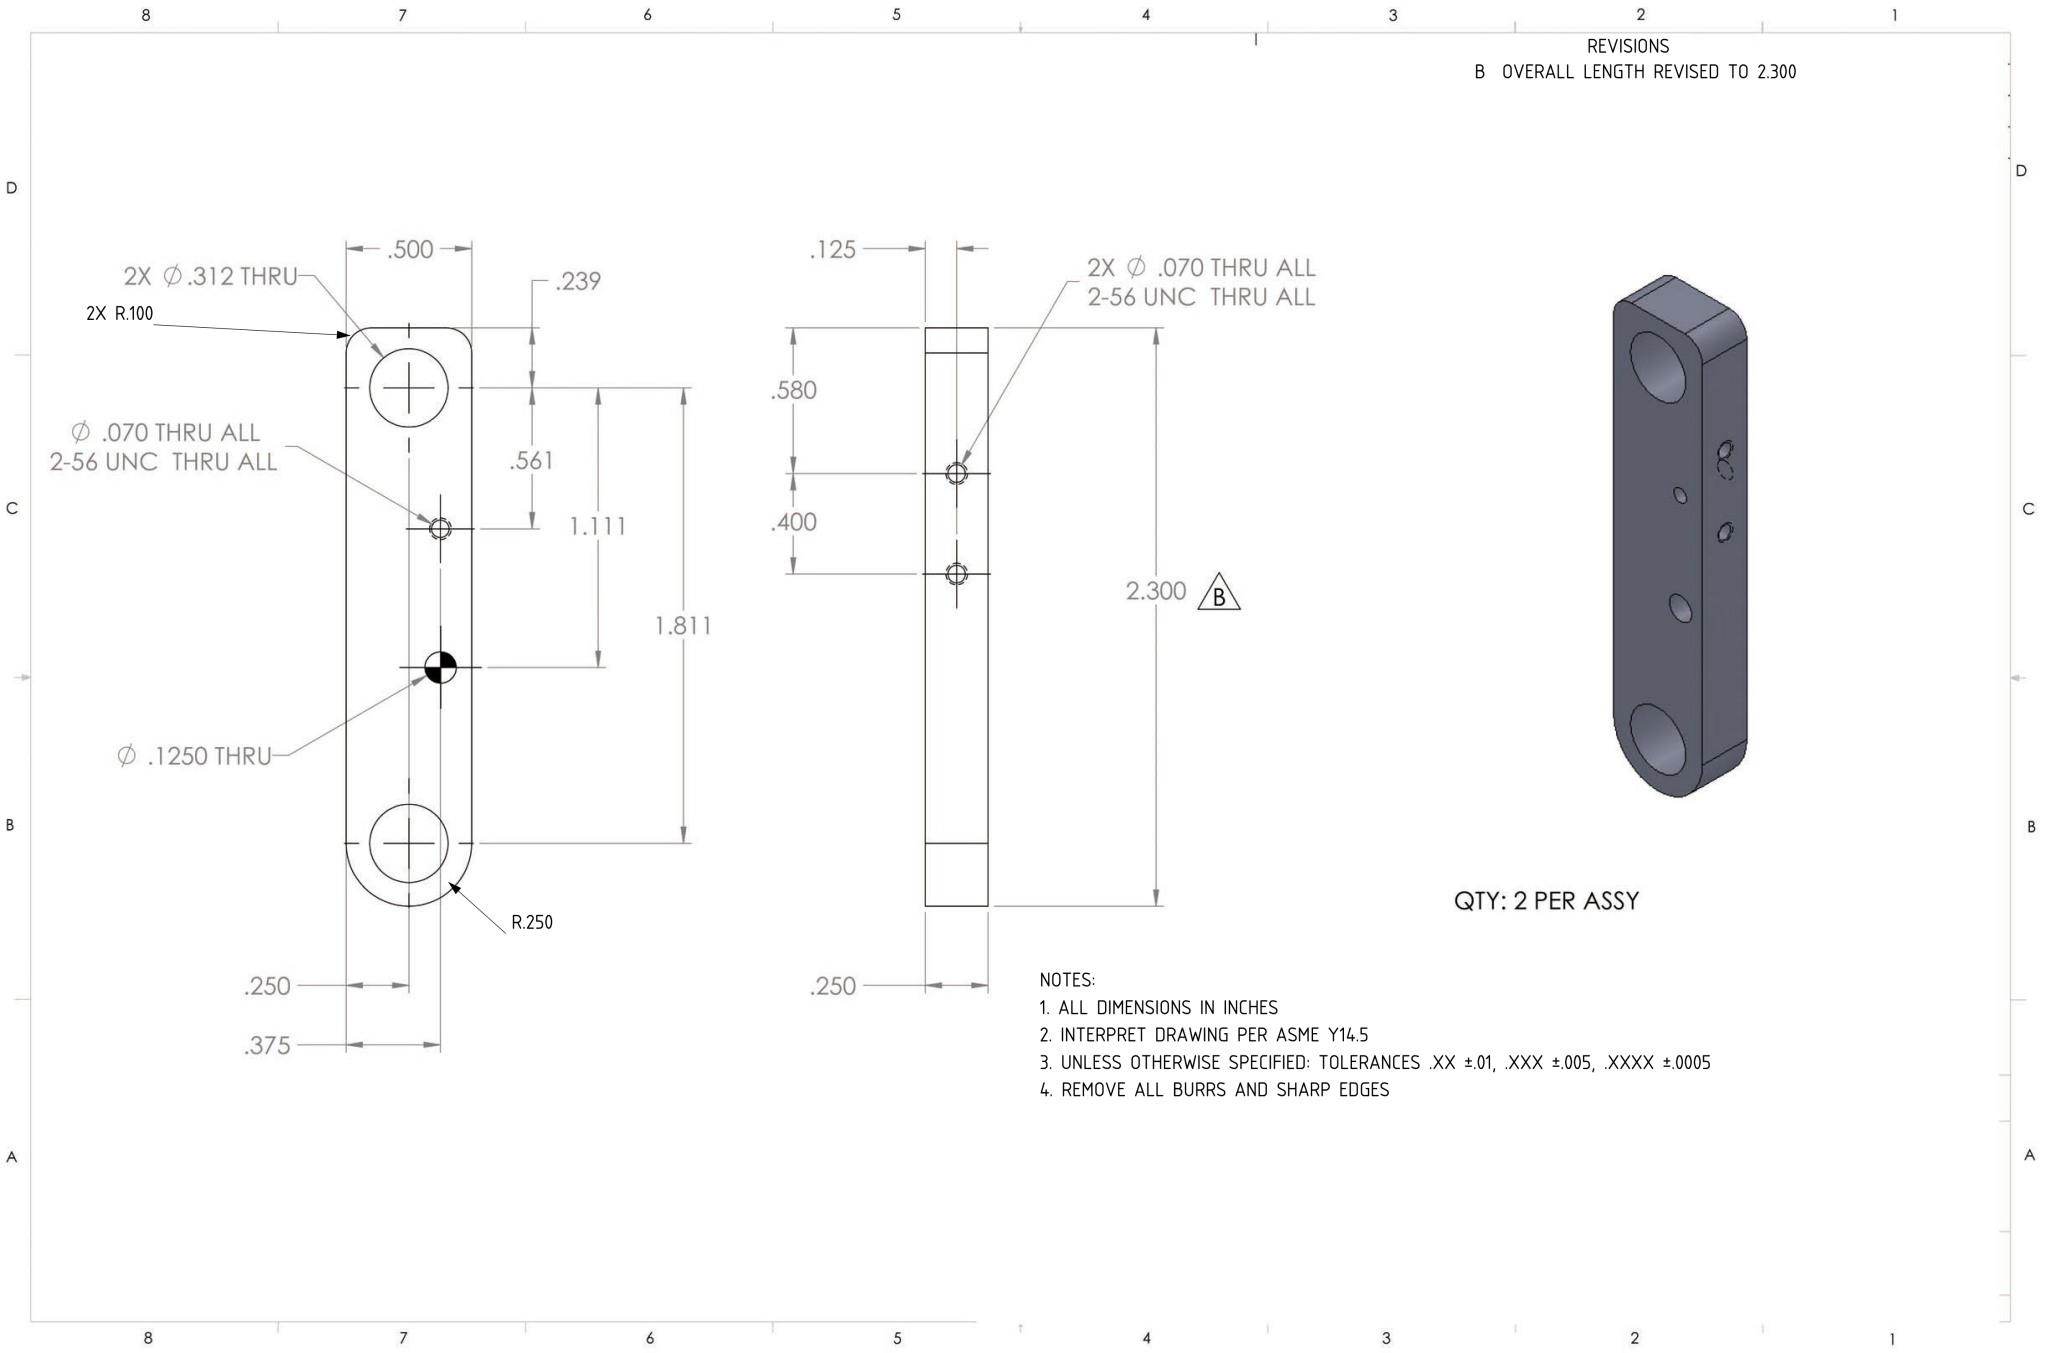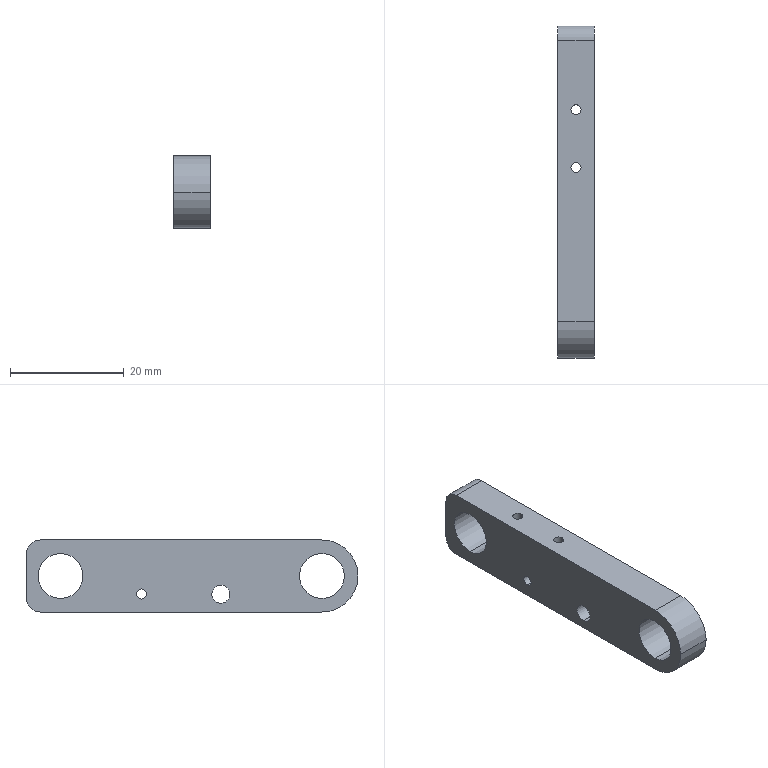Part | NX | drawing in inches | 1 solid | 21 faces | box 6.35 x 58.42 x 12.7 mm | volume 3828 mm3 | cylinder 16 | plane 5 | commonest cylinder face diameters 1.778 x6 7.925 x4 3.175 x2 5.08 x2 12.7 x2
STEP:
#1=COLOUR_RGB('',0.7922,0.8196,0.9333);
#2=FILL_AREA_STYLE_COLOUR('',#1);
#3=FILL_AREA_STYLE('',(#2));
#4=SURFACE_STYLE_FILL_AREA(#3);
#5=SURFACE_SIDE_STYLE('',(#4));
#6=SURFACE_STYLE_USAGE(.BOTH.,#5);
#7=PRESENTATION_STYLE_ASSIGNMENT((#6));
#8=CARTESIAN_POINT('',(-0.09,1.47,0.25));
#9=VERTEX_POINT('',#8);
#10=CARTESIAN_POINT('',(-0.09,1.47,-0.25));
#11=VERTEX_POINT('',#10);
#12=CARTESIAN_POINT('',(-0.09,1.47,-0.25));
#13=DIRECTION('',(0.,0.,-1.));
#14=VECTOR('',#13,39.37);
#15=LINE('',#12,#14);
#16=EDGE_CURVE('',#9,#11,#15,.T.);
#17=ORIENTED_EDGE('',*,*,#16,.F.);
#18=CARTESIAN_POINT('',(-0.16,1.47,0.25));
#19=VERTEX_POINT('',#18);
#20=CARTESIAN_POINT('',(-0.125,1.47,0.25));
#21=DIRECTION('',(0.,0.,-1.));
#22=DIRECTION('',(-1.,0.,0.));
#23=AXIS2_PLACEMENT_3D('',#20,#21,#22);
#24=CIRCLE('',#23,0.035);
#25=EDGE_CURVE('',#19,#9,#24,.T.);
#26=ORIENTED_EDGE('',*,*,#25,.F.);
#27=CARTESIAN_POINT('',(-0.16,1.47,-0.25));
#28=VERTEX_POINT('',#27);
#29=CARTESIAN_POINT('',(-0.16,1.47,-0.25));
#30=DIRECTION('',(0.,0.,-1.));
#31=VECTOR('',#30,39.37);
#32=LINE('',#29,#31);
#33=EDGE_CURVE('',#19,#28,#32,.T.);
#34=ORIENTED_EDGE('',*,*,#33,.T.);
#35=CARTESIAN_POINT('',(-0.125,1.47,-0.25));
#36=DIRECTION('',(0.,0.,-1.));
#37=DIRECTION('',(-1.,0.,0.));
#38=AXIS2_PLACEMENT_3D('',#35,#36,#37);
#39=CIRCLE('',#38,0.035);
#40=EDGE_CURVE('',#28,#11,#39,.T.);
#41=ORIENTED_EDGE('',*,*,#40,.T.);
#42=EDGE_LOOP('',(#17,#26,#34,#41));
#43=FACE_OUTER_BOUND('',#42,.T.);
#44=CARTESIAN_POINT('',(-0.125,1.47,-0.25));
#45=DIRECTION('',(0.,0.,-1.));
#46=DIRECTION('',(-1.,0.,0.));
#47=AXIS2_PLACEMENT_3D('',#44,#45,#46);
#48=CYLINDRICAL_SURFACE('',#47,0.035);
#49=ADVANCED_FACE('',(#43),#48,.F.);
#50=STYLED_ITEM('',(#7),#49);
#51=PRESENTATION_LAYER_ASSIGNMENT('','',(#50));
#52=COLOUR_RGB('',0.7922,0.8196,0.9333);
#53=FILL_AREA_STYLE_COLOUR('',#52);
#54=FILL_AREA_STYLE('',(#53));
#55=SURFACE_STYLE_FILL_AREA(#54);
#56=SURFACE_SIDE_STYLE('',(#55));
#57=SURFACE_STYLE_USAGE(.BOTH.,#56);
#58=PRESENTATION_STYLE_ASSIGNMENT((#57));
#59=CARTESIAN_POINT('',(0.,1.25,-0.16));
#60=VERTEX_POINT('',#59);
#61=CARTESIAN_POINT('',(0.,1.25,-0.09));
#62=VERTEX_POINT('',#61);
#63=CARTESIAN_POINT('',(0.,1.25,-0.125));
#64=DIRECTION('',(-1.,0.,0.));
#65=DIRECTION('',(0.,0.,1.));
#66=AXIS2_PLACEMENT_3D('',#63,#64,#65);
#67=CIRCLE('',#66,0.035);
#68=EDGE_CURVE('',#60,#62,#67,.T.);
#69=ORIENTED_EDGE('',*,*,#68,.F.);
#70=CARTESIAN_POINT('',(-0.25,1.25,-0.16));
#71=VERTEX_POINT('',#70);
#72=CARTESIAN_POINT('',(-0.25,1.25,-0.16));
#73=DIRECTION('',(-1.,0.,0.));
#74=VECTOR('',#73,39.37);
#75=LINE('',#72,#74);
#76=EDGE_CURVE('',#60,#71,#75,.T.);
#77=ORIENTED_EDGE('',*,*,#76,.T.);
#78=CARTESIAN_POINT('',(-0.25,1.25,-0.09));
#79=VERTEX_POINT('',#78);
#80=CARTESIAN_POINT('',(-0.25,1.25,-0.125));
#81=DIRECTION('',(-1.,0.,0.));
#82=DIRECTION('',(0.,0.,1.));
#83=AXIS2_PLACEMENT_3D('',#80,#81,#82);
#84=CIRCLE('',#83,0.035);
#85=EDGE_CURVE('',#71,#79,#84,.T.);
#86=ORIENTED_EDGE('',*,*,#85,.T.);
#87=CARTESIAN_POINT('',(-0.25,1.25,-0.09));
#88=DIRECTION('',(-1.,0.,0.));
#89=VECTOR('',#88,39.37);
#90=LINE('',#87,#89);
#91=EDGE_CURVE('',#62,#79,#90,.T.);
#92=ORIENTED_EDGE('',*,*,#91,.F.);
#93=EDGE_LOOP('',(#69,#77,#86,#92));
#94=FACE_OUTER_BOUND('',#93,.T.);
#95=CARTESIAN_POINT('',(-0.25,1.25,-0.125));
#96=DIRECTION('',(-1.,0.,0.));
#97=DIRECTION('',(0.,0.,1.));
#98=AXIS2_PLACEMENT_3D('',#95,#96,#97);
#99=CYLINDRICAL_SURFACE('',#98,0.035);
#100=ADVANCED_FACE('',(#94),#99,.F.);
#101=CARTESIAN_POINT('',(-0.25,0.7,-0.1886));
#102=VERTEX_POINT('',#101);
#103=CARTESIAN_POINT('',(-0.25,0.7,-0.06365));
#104=VERTEX_POINT('',#103);
#105=CARTESIAN_POINT('',(-0.25,0.7,-0.1261));
#106=DIRECTION('',(-1.,0.,0.));
#107=DIRECTION('',(0.,0.,1.));
#108=AXIS2_PLACEMENT_3D('',#105,#106,#107);
#109=CIRCLE('',#108,0.0625);
#110=EDGE_CURVE('',#102,#104,#109,.T.);
#111=ORIENTED_EDGE('',*,*,#110,.T.);
#112=CARTESIAN_POINT('',(0.,0.7,-0.06365));
#113=VERTEX_POINT('',#112);
#114=CARTESIAN_POINT('',(0.,0.7,-0.06365));
#115=DIRECTION('',(1.,0.,0.));
#116=VECTOR('',#115,39.37);
#117=LINE('',#114,#116);
#118=EDGE_CURVE('',#104,#113,#117,.T.);
#119=ORIENTED_EDGE('',*,*,#118,.T.);
#120=CARTESIAN_POINT('',(0.,0.7,-0.1886));
#121=VERTEX_POINT('',#120);
#122=CARTESIAN_POINT('',(0.,0.7,-0.1261));
#123=DIRECTION('',(1.,0.,0.));
#124=DIRECTION('',(0.,0.,-1.));
#125=AXIS2_PLACEMENT_3D('',#122,#123,#124);
#126=CIRCLE('',#125,0.0625);
#127=EDGE_CURVE('',#113,#121,#126,.T.);
#128=ORIENTED_EDGE('',*,*,#127,.T.);
#129=CARTESIAN_POINT('',(0.,0.7,-0.1886));
#130=DIRECTION('',(1.,0.,0.));
#131=VECTOR('',#130,39.37);
#132=LINE('',#129,#131);
#133=EDGE_CURVE('',#102,#121,#132,.T.);
#134=ORIENTED_EDGE('',*,*,#133,.F.);
#135=EDGE_LOOP('',(#111,#119,#128,#134));
#136=FACE_OUTER_BOUND('',#135,.T.);
#137=CARTESIAN_POINT('',(0.,0.7,-0.1261));
#138=DIRECTION('',(1.,0.,0.));
#139=DIRECTION('',(0.,0.,-1.));
#140=AXIS2_PLACEMENT_3D('',#137,#138,#139);
#141=CYLINDRICAL_SURFACE('',#140,0.0625);
#142=ADVANCED_FACE('',(#136),#141,.F.);
#143=CARTESIAN_POINT('',(-0.125,1.47,0.25));
#144=DIRECTION('',(0.,0.,-1.));
#145=DIRECTION('',(-1.,0.,0.));
#146=AXIS2_PLACEMENT_3D('',#143,#144,#145);
#147=CIRCLE('',#146,0.035);
#148=EDGE_CURVE('',#9,#19,#147,.T.);
#149=ORIENTED_EDGE('',*,*,#148,.F.);
#150=ORIENTED_EDGE('',*,*,#16,.T.);
#151=CARTESIAN_POINT('',(-0.125,1.47,-0.25));
#152=DIRECTION('',(0.,0.,-1.));
#153=DIRECTION('',(-1.,0.,0.));
#154=AXIS2_PLACEMENT_3D('',#151,#152,#153);
#155=CIRCLE('',#154,0.035);
#156=EDGE_CURVE('',#11,#28,#155,.T.);
#157=ORIENTED_EDGE('',*,*,#156,.T.);
#158=ORIENTED_EDGE('',*,*,#33,.F.);
#159=EDGE_LOOP('',(#149,#150,#157,#158));
#160=FACE_OUTER_BOUND('',#159,.T.);
#161=CARTESIAN_POINT('',(-0.125,1.47,-0.25));
#162=DIRECTION('',(0.,0.,-1.));
#163=DIRECTION('',(-1.,0.,0.));
#164=AXIS2_PLACEMENT_3D('',#161,#162,#163);
#165=CYLINDRICAL_SURFACE('',#164,0.035);
#166=ADVANCED_FACE('',(#160),#165,.F.);
#167=CARTESIAN_POINT('',(-0.09,1.07,0.25));
#168=VERTEX_POINT('',#167);
#169=CARTESIAN_POINT('',(-0.16,1.07,0.25));
#170=VERTEX_POINT('',#169);
#171=CARTESIAN_POINT('',(-0.125,1.07,0.25));
#172=DIRECTION('',(0.,0.,-1.));
#173=DIRECTION('',(-1.,0.,0.));
#174=AXIS2_PLACEMENT_3D('',#171,#172,#173);
#175=CIRCLE('',#174,0.035);
#176=EDGE_CURVE('',#168,#170,#175,.T.);
#177=ORIENTED_EDGE('',*,*,#176,.F.);
#178=CARTESIAN_POINT('',(-0.09,1.07,-0.25));
#179=VERTEX_POINT('',#178);
#180=CARTESIAN_POINT('',(-0.09,1.07,-0.25));
#181=DIRECTION('',(0.,0.,-1.));
#182=VECTOR('',#181,39.37);
#183=LINE('',#180,#182);
#184=EDGE_CURVE('',#168,#179,#183,.T.);
#185=ORIENTED_EDGE('',*,*,#184,.T.);
#186=CARTESIAN_POINT('',(-0.16,1.07,-0.25));
#187=VERTEX_POINT('',#186);
#188=CARTESIAN_POINT('',(-0.125,1.07,-0.25));
#189=DIRECTION('',(0.,0.,-1.));
#190=DIRECTION('',(-1.,0.,0.));
#191=AXIS2_PLACEMENT_3D('',#188,#189,#190);
#192=CIRCLE('',#191,0.035);
#193=EDGE_CURVE('',#179,#187,#192,.T.);
#194=ORIENTED_EDGE('',*,*,#193,.T.);
#195=CARTESIAN_POINT('',(-0.16,1.07,-0.25));
#196=DIRECTION('',(0.,0.,-1.));
#197=VECTOR('',#196,39.37);
#198=LINE('',#195,#197);
#199=EDGE_CURVE('',#170,#187,#198,.T.);
#200=ORIENTED_EDGE('',*,*,#199,.F.);
#201=EDGE_LOOP('',(#177,#185,#194,#200));
#202=FACE_OUTER_BOUND('',#201,.T.);
#203=CARTESIAN_POINT('',(-0.125,1.07,-0.25));
#204=DIRECTION('',(0.,0.,-1.));
#205=DIRECTION('',(-1.,0.,0.));
#206=AXIS2_PLACEMENT_3D('',#203,#204,#205);
#207=CYLINDRICAL_SURFACE('',#206,0.035);
#208=ADVANCED_FACE('',(#202),#207,.F.);
#209=CARTESIAN_POINT('',(-0.25,1.811,0.156));
#210=VERTEX_POINT('',#209);
#211=CARTESIAN_POINT('',(-0.25,1.811,-0.156));
#212=VERTEX_POINT('',#211);
#213=CARTESIAN_POINT('',(-0.25,1.811,0.));
#214=DIRECTION('',(1.,0.,0.));
#215=DIRECTION('',(0.,0.,1.));
#216=AXIS2_PLACEMENT_3D('',#213,#214,#215);
#217=CIRCLE('',#216,0.156);
#218=EDGE_CURVE('',#210,#212,#217,.T.);
#219=ORIENTED_EDGE('',*,*,#218,.F.);
#220=CARTESIAN_POINT('',(0.,1.811,0.156));
#221=VERTEX_POINT('',#220);
#222=CARTESIAN_POINT('',(-0.25,1.811,0.156));
#223=DIRECTION('',(1.,0.,0.));
#224=VECTOR('',#223,39.37);
#225=LINE('',#222,#224);
#226=EDGE_CURVE('',#210,#221,#225,.T.);
#227=ORIENTED_EDGE('',*,*,#226,.T.);
#228=CARTESIAN_POINT('',(0.,1.811,-0.156));
#229=VERTEX_POINT('',#228);
#230=CARTESIAN_POINT('',(0.,1.811,0.));
#231=DIRECTION('',(1.,0.,0.));
#232=DIRECTION('',(0.,0.,-1.));
#233=AXIS2_PLACEMENT_3D('',#230,#231,#232);
#234=CIRCLE('',#233,0.156);
#235=EDGE_CURVE('',#221,#229,#234,.T.);
#236=ORIENTED_EDGE('',*,*,#235,.T.);
#237=CARTESIAN_POINT('',(-0.25,1.811,-0.156));
#238=DIRECTION('',(1.,0.,0.));
#239=VECTOR('',#238,39.37);
#240=LINE('',#237,#239);
#241=EDGE_CURVE('',#212,#229,#240,.T.);
#242=ORIENTED_EDGE('',*,*,#241,.F.);
#243=EDGE_LOOP('',(#219,#227,#236,#242));
#244=FACE_OUTER_BOUND('',#243,.T.);
#245=CARTESIAN_POINT('',(-0.25,1.811,0.));
#246=DIRECTION('',(1.,0.,0.));
#247=DIRECTION('',(0.,0.,-1.));
#248=AXIS2_PLACEMENT_3D('',#245,#246,#247);
#249=CYLINDRICAL_SURFACE('',#248,0.156);
#250=ADVANCED_FACE('',(#244),#249,.F.);
#251=CARTESIAN_POINT('',(-0.25,0.,0.156));
#252=VERTEX_POINT('',#251);
#253=CARTESIAN_POINT('',(-0.25,0.,-0.156));
#254=VERTEX_POINT('',#253);
#255=CARTESIAN_POINT('',(-0.25,0.,0.));
#256=DIRECTION('',(1.,0.,0.));
#257=DIRECTION('',(0.,0.,1.));
#258=AXIS2_PLACEMENT_3D('',#255,#256,#257);
#259=CIRCLE('',#258,0.156);
#260=EDGE_CURVE('',#252,#254,#259,.T.);
#261=ORIENTED_EDGE('',*,*,#260,.F.);
#262=CARTESIAN_POINT('',(0.,0.,0.156));
#263=VERTEX_POINT('',#262);
#264=CARTESIAN_POINT('',(-0.25,0.,0.156));
#265=DIRECTION('',(1.,0.,0.));
#266=VECTOR('',#265,39.37);
#267=LINE('',#264,#266);
#268=EDGE_CURVE('',#252,#263,#267,.T.);
#269=ORIENTED_EDGE('',*,*,#268,.T.);
#270=CARTESIAN_POINT('',(0.,0.,-0.156));
#271=VERTEX_POINT('',#270);
#272=CARTESIAN_POINT('',(0.,0.,0.));
#273=DIRECTION('',(1.,0.,0.));
#274=DIRECTION('',(0.,0.,-1.));
#275=AXIS2_PLACEMENT_3D('',#272,#273,#274);
#276=CIRCLE('',#275,0.156);
#277=EDGE_CURVE('',#263,#271,#276,.T.);
#278=ORIENTED_EDGE('',*,*,#277,.T.);
#279=CARTESIAN_POINT('',(-0.25,0.,-0.156));
#280=DIRECTION('',(1.,0.,0.));
#281=VECTOR('',#280,39.37);
#282=LINE('',#279,#281);
#283=EDGE_CURVE('',#254,#271,#282,.T.);
#284=ORIENTED_EDGE('',*,*,#283,.F.);
#285=EDGE_LOOP('',(#261,#269,#278,#284));
#286=FACE_OUTER_BOUND('',#285,.T.);
#287=CARTESIAN_POINT('',(-0.25,0.,0.));
#288=DIRECTION('',(1.,0.,0.));
#289=DIRECTION('',(0.,0.,-1.));
#290=AXIS2_PLACEMENT_3D('',#287,#288,#289);
#291=CYLINDRICAL_SURFACE('',#290,0.156);
#292=ADVANCED_FACE('',(#286),#291,.F.);
#293=ORIENTED_EDGE('',*,*,#25,.T.);
#294=ORIENTED_EDGE('',*,*,#148,.T.);
#295=EDGE_LOOP('',(#293,#294));
#296=FACE_BOUND('',#295,.T.);
#297=CARTESIAN_POINT('',(-0.125,1.07,0.25));
#298=DIRECTION('',(0.,0.,-1.));
#299=DIRECTION('',(-1.,0.,0.));
#300=AXIS2_PLACEMENT_3D('',#297,#298,#299);
#301=CIRCLE('',#300,0.035);
#302=EDGE_CURVE('',#170,#168,#301,.T.);
#303=ORIENTED_EDGE('',*,*,#302,.T.);
#304=ORIENTED_EDGE('',*,*,#176,.T.);
#305=EDGE_LOOP('',(#303,#304));
#306=FACE_BOUND('',#305,.T.);
#307=CARTESIAN_POINT('',(-0.25,1.95,0.25));
#308=VERTEX_POINT('',#307);
#309=CARTESIAN_POINT('',(-0.25,-0.,0.25));
#310=VERTEX_POINT('',#309);
#311=CARTESIAN_POINT('',(-0.25,-0.25,0.25));
#312=DIRECTION('',(0.,-1.,-0.));
#313=VECTOR('',#312,39.37);
#314=LINE('',#311,#313);
#315=EDGE_CURVE('',#308,#310,#314,.T.);
#316=ORIENTED_EDGE('',*,*,#315,.T.);
#317=CARTESIAN_POINT('',(0.,-0.,0.25));
#318=VERTEX_POINT('',#317);
#319=CARTESIAN_POINT('',(-0.25,-0.,0.25));
#320=DIRECTION('',(1.,0.,0.));
#321=VECTOR('',#320,39.37);
#322=LINE('',#319,#321);
#323=EDGE_CURVE('',#310,#318,#322,.T.);
#324=ORIENTED_EDGE('',*,*,#323,.T.);
#325=CARTESIAN_POINT('',(0.,1.95,0.25));
#326=VERTEX_POINT('',#325);
#327=CARTESIAN_POINT('',(0.,-0.25,0.25));
#328=DIRECTION('',(0.,-1.,-0.));
#329=VECTOR('',#328,39.37);
#330=LINE('',#327,#329);
#331=EDGE_CURVE('',#326,#318,#330,.T.);
#332=ORIENTED_EDGE('',*,*,#331,.F.);
#333=CARTESIAN_POINT('',(-0.25,1.95,0.25));
#334=DIRECTION('',(-1.,0.,0.));
#335=VECTOR('',#334,39.37);
#336=LINE('',#333,#335);
#337=EDGE_CURVE('',#326,#308,#336,.T.);
#338=ORIENTED_EDGE('',*,*,#337,.T.);
#339=EDGE_LOOP('',(#316,#324,#332,#338));
#340=FACE_OUTER_BOUND('',#339,.T.);
#341=CARTESIAN_POINT('',(-0.25,-0.25,0.25));
#342=DIRECTION('',(0.,-0.,1.));
#343=DIRECTION('',(0.,-1.,-0.));
#344=AXIS2_PLACEMENT_3D('',#341,#342,#343);
#345=PLANE('',#344);
#346=ADVANCED_FACE('',(#296,#306,#340),#345,.T.);
#347=CARTESIAN_POINT('',(-0.25,2.05,-0.15));
#348=VERTEX_POINT('',#347);
#349=CARTESIAN_POINT('',(-0.25,2.05,0.15));
#350=VERTEX_POINT('',#349);
#351=CARTESIAN_POINT('',(-0.25,2.05,0.25));
#352=DIRECTION('',(0.,0.,1.));
#353=VECTOR('',#352,39.37);
#354=LINE('',#351,#353);
#355=EDGE_CURVE('',#348,#350,#354,.T.);
#356=ORIENTED_EDGE('',*,*,#355,.T.);
#357=CARTESIAN_POINT('',(0.,2.05,0.15));
#358=VERTEX_POINT('',#357);
#359=CARTESIAN_POINT('',(-0.25,2.05,0.15));
#360=DIRECTION('',(1.,0.,0.));
#361=VECTOR('',#360,39.37);
#362=LINE('',#359,#361);
#363=EDGE_CURVE('',#350,#358,#362,.T.);
#364=ORIENTED_EDGE('',*,*,#363,.T.);
#365=CARTESIAN_POINT('',(0.,2.05,-0.15));
#366=VERTEX_POINT('',#365);
#367=CARTESIAN_POINT('',(0.,2.05,0.25));
#368=DIRECTION('',(0.,0.,1.));
#369=VECTOR('',#368,39.37);
#370=LINE('',#367,#369);
#371=EDGE_CURVE('',#366,#358,#370,.T.);
#372=ORIENTED_EDGE('',*,*,#371,.F.);
#373=CARTESIAN_POINT('',(-0.25,2.05,-0.15));
#374=DIRECTION('',(-1.,0.,0.));
#375=VECTOR('',#374,39.37);
#376=LINE('',#373,#375);
#377=EDGE_CURVE('',#366,#348,#376,.T.);
#378=ORIENTED_EDGE('',*,*,#377,.T.);
#379=EDGE_LOOP('',(#356,#364,#372,#378));
#380=FACE_OUTER_BOUND('',#379,.T.);
#381=CARTESIAN_POINT('',(-0.25,2.05,0.25));
#382=DIRECTION('',(0.,1.,0.));
#383=DIRECTION('',(0.,0.,1.));
#384=AXIS2_PLACEMENT_3D('',#381,#382,#383);
#385=PLANE('',#384);
#386=ADVANCED_FACE('',(#380),#385,.T.);
#387=ORIENTED_EDGE('',*,*,#40,.F.);
#388=ORIENTED_EDGE('',*,*,#156,.F.);
#389=EDGE_LOOP('',(#387,#388));
#390=FACE_BOUND('',#389,.T.);
#391=CARTESIAN_POINT('',(-0.125,1.07,-0.25));
#392=DIRECTION('',(0.,0.,-1.));
#393=DIRECTION('',(-1.,0.,0.));
#394=AXIS2_PLACEMENT_3D('',#391,#392,#393);
#395=CIRCLE('',#394,0.035);
#396=EDGE_CURVE('',#187,#179,#395,.T.);
#397=ORIENTED_EDGE('',*,*,#396,.F.);
#398=ORIENTED_EDGE('',*,*,#193,.F.);
#399=EDGE_LOOP('',(#397,#398));
#400=FACE_BOUND('',#399,.T.);
#401=CARTESIAN_POINT('',(0.,0.,-0.25));
#402=VERTEX_POINT('',#401);
#403=CARTESIAN_POINT('',(0.,1.95,-0.25));
#404=VERTEX_POINT('',#403);
#405=CARTESIAN_POINT('',(0.,-0.25,-0.25));
#406=DIRECTION('',(0.,1.,0.));
#407=VECTOR('',#406,39.37);
#408=LINE('',#405,#407);
#409=EDGE_CURVE('',#402,#404,#408,.T.);
#410=ORIENTED_EDGE('',*,*,#409,.F.);
#411=CARTESIAN_POINT('',(-0.25,0.,-0.25));
#412=VERTEX_POINT('',#411);
#413=CARTESIAN_POINT('',(-0.25,0.,-0.25));
#414=DIRECTION('',(-1.,0.,0.));
#415=VECTOR('',#414,39.37);
#416=LINE('',#413,#415);
#417=EDGE_CURVE('',#402,#412,#416,.T.);
#418=ORIENTED_EDGE('',*,*,#417,.T.);
#419=CARTESIAN_POINT('',(-0.25,1.95,-0.25));
#420=VERTEX_POINT('',#419);
#421=CARTESIAN_POINT('',(-0.25,-0.25,-0.25));
#422=DIRECTION('',(0.,1.,0.));
#423=VECTOR('',#422,39.37);
#424=LINE('',#421,#423);
#425=EDGE_CURVE('',#412,#420,#424,.T.);
#426=ORIENTED_EDGE('',*,*,#425,.T.);
#427=CARTESIAN_POINT('',(-0.25,1.95,-0.25));
#428=DIRECTION('',(1.,0.,0.));
#429=VECTOR('',#428,39.37);
#430=LINE('',#427,#429);
#431=EDGE_CURVE('',#420,#404,#430,.T.);
#432=ORIENTED_EDGE('',*,*,#431,.T.);
#433=EDGE_LOOP('',(#410,#418,#426,#432));
#434=FACE_OUTER_BOUND('',#433,.T.);
#435=CARTESIAN_POINT('',(-0.25,-0.25,-0.25));
#436=DIRECTION('',(0.,0.,-1.));
#437=DIRECTION('',(-1.,0.,0.));
#438=AXIS2_PLACEMENT_3D('',#435,#436,#437);
#439=PLANE('',#438);
#440=ADVANCED_FACE('',(#390,#400,#434),#439,.T.);
#441=CARTESIAN_POINT('',(-0.25,1.25,-0.125));
#442=DIRECTION('',(-1.,0.,0.));
#443=DIRECTION('',(0.,0.,1.));
#444=AXIS2_PLACEMENT_3D('',#441,#442,#443);
#445=CIRCLE('',#444,0.035);
#446=EDGE_CURVE('',#79,#71,#445,.T.);
#447=ORIENTED_EDGE('',*,*,#446,.F.);
#448=ORIENTED_EDGE('',*,*,#85,.F.);
#449=EDGE_LOOP('',(#447,#448));
#450=FACE_BOUND('',#449,.T.);
#451=ORIENTED_EDGE('',*,*,#110,.F.);
#452=CARTESIAN_POINT('',(-0.25,0.7,-0.1261));
#453=DIRECTION('',(-1.,0.,0.));
#454=DIRECTION('',(0.,0.,1.));
#455=AXIS2_PLACEMENT_3D('',#452,#453,#454);
#456=CIRCLE('',#455,0.0625);
#457=EDGE_CURVE('',#104,#102,#456,.T.);
#458=ORIENTED_EDGE('',*,*,#457,.F.);
#459=EDGE_LOOP('',(#451,#458));
#460=FACE_BOUND('',#459,.T.);
#461=CARTESIAN_POINT('',(-0.25,1.811,0.));
#462=DIRECTION('',(1.,0.,0.));
#463=DIRECTION('',(0.,0.,1.));
#464=AXIS2_PLACEMENT_3D('',#461,#462,#463);
#465=CIRCLE('',#464,0.156);
#466=EDGE_CURVE('',#212,#210,#465,.T.);
#467=ORIENTED_EDGE('',*,*,#466,.T.);
#468=ORIENTED_EDGE('',*,*,#218,.T.);
#469=EDGE_LOOP('',(#467,#468));
#470=FACE_BOUND('',#469,.T.);
#471=CARTESIAN_POINT('',(-0.25,0.,0.));
#472=DIRECTION('',(1.,0.,0.));
#473=DIRECTION('',(0.,0.,1.));
#474=AXIS2_PLACEMENT_3D('',#471,#472,#473);
#475=CIRCLE('',#474,0.156);
#476=EDGE_CURVE('',#254,#252,#475,.T.);
#477=ORIENTED_EDGE('',*,*,#476,.T.);
#478=ORIENTED_EDGE('',*,*,#260,.T.);
#479=EDGE_LOOP('',(#477,#478));
#480=FACE_BOUND('',#479,.T.);
#481=ORIENTED_EDGE('',*,*,#425,.F.);
#482=CARTESIAN_POINT('',(-0.25,-0.25,0.));
#483=VERTEX_POINT('',#482);
#484=CARTESIAN_POINT('',(-0.25,0.,-0.));
#485=DIRECTION('',(-1.,0.,0.));
#486=DIRECTION('',(0.,0.,1.));
#487=AXIS2_PLACEMENT_3D('',#484,#485,#486);
#488=CIRCLE('',#487,0.25);
#489=EDGE_CURVE('',#412,#483,#488,.T.);
#490=ORIENTED_EDGE('',*,*,#489,.T.);
#491=CARTESIAN_POINT('',(-0.25,0.,0.));
#492=DIRECTION('',(-1.,0.,0.));
#493=DIRECTION('',(0.,0.,1.));
#494=AXIS2_PLACEMENT_3D('',#491,#492,#493);
#495=CIRCLE('',#494,0.25);
#496=EDGE_CURVE('',#483,#310,#495,.T.);
#497=ORIENTED_EDGE('',*,*,#496,.T.);
#498=ORIENTED_EDGE('',*,*,#315,.F.);
#499=CARTESIAN_POINT('',(-0.25,1.95,0.15));
#500=DIRECTION('',(-1.,0.,0.));
#501=DIRECTION('',(0.,0.,1.));
#502=AXIS2_PLACEMENT_3D('',#499,#500,#501);
#503=CIRCLE('',#502,0.1);
#504=EDGE_CURVE('',#308,#350,#503,.T.);
#505=ORIENTED_EDGE('',*,*,#504,.T.);
#506=ORIENTED_EDGE('',*,*,#355,.F.);
#507=CARTESIAN_POINT('',(-0.25,1.95,-0.15));
#508=DIRECTION('',(-1.,0.,0.));
#509=DIRECTION('',(0.,0.,1.));
#510=AXIS2_PLACEMENT_3D('',#507,#508,#509);
#511=CIRCLE('',#510,0.1);
#512=EDGE_CURVE('',#348,#420,#511,.T.);
#513=ORIENTED_EDGE('',*,*,#512,.T.);
#514=EDGE_LOOP('',(#481,#490,#497,#498,#505,#506,#513));
#515=FACE_OUTER_BOUND('',#514,.T.);
#516=CARTESIAN_POINT('',(-0.25,0.,0.));
#517=DIRECTION('',(-1.,0.,0.));
#518=DIRECTION('',(0.,0.,1.));
#519=AXIS2_PLACEMENT_3D('',#516,#517,#518);
#520=PLANE('',#519);
#521=ADVANCED_FACE('',(#450,#460,#470,#480,#515),#520,.T.);
#522=CARTESIAN_POINT('',(0.,1.25,-0.125));
#523=DIRECTION('',(-1.,0.,0.));
#524=DIRECTION('',(0.,0.,1.));
#525=AXIS2_PLACEMENT_3D('',#522,#523,#524);
#526=CIRCLE('',#525,0.035);
#527=EDGE_CURVE('',#62,#60,#526,.T.);
#528=ORIENTED_EDGE('',*,*,#527,.T.);
#529=ORIENTED_EDGE('',*,*,#68,.T.);
#530=EDGE_LOOP('',(#528,#529));
#531=FACE_BOUND('',#530,.T.);
#532=CARTESIAN_POINT('',(0.,0.7,-0.1261));
#533=DIRECTION('',(1.,0.,0.));
#534=DIRECTION('',(0.,0.,-1.));
#535=AXIS2_PLACEMENT_3D('',#532,#533,#534);
#536=CIRCLE('',#535,0.0625);
#537=EDGE_CURVE('',#121,#113,#536,.T.);
#538=ORIENTED_EDGE('',*,*,#537,.F.);
#539=ORIENTED_EDGE('',*,*,#127,.F.);
#540=EDGE_LOOP('',(#538,#539));
#541=FACE_BOUND('',#540,.T.);
#542=CARTESIAN_POINT('',(0.,1.811,0.));
#543=DIRECTION('',(1.,0.,0.));
#544=DIRECTION('',(0.,0.,-1.));
#545=AXIS2_PLACEMENT_3D('',#542,#543,#544);
#546=CIRCLE('',#545,0.156);
#547=EDGE_CURVE('',#229,#221,#546,.T.);
#548=ORIENTED_EDGE('',*,*,#547,.F.);
#549=ORIENTED_EDGE('',*,*,#235,.F.);
#550=EDGE_LOOP('',(#548,#549));
#551=FACE_BOUND('',#550,.T.);
#552=CARTESIAN_POINT('',(0.,0.,0.));
#553=DIRECTION('',(1.,0.,0.));
#554=DIRECTION('',(0.,0.,-1.));
#555=AXIS2_PLACEMENT_3D('',#552,#553,#554);
#556=CIRCLE('',#555,0.156);
#557=EDGE_CURVE('',#271,#263,#556,.T.);
#558=ORIENTED_EDGE('',*,*,#557,.F.);
#559=ORIENTED_EDGE('',*,*,#277,.F.);
#560=EDGE_LOOP('',(#558,#559));
#561=FACE_BOUND('',#560,.T.);
#562=CARTESIAN_POINT('',(0.,-0.25,0.));
#563=VERTEX_POINT('',#562);
#564=CARTESIAN_POINT('',(0.,0.,0.));
#565=DIRECTION('',(1.,0.,0.));
#566=DIRECTION('',(0.,0.,1.));
#567=AXIS2_PLACEMENT_3D('',#564,#565,#566);
#568=CIRCLE('',#567,0.25);
#569=EDGE_CURVE('',#318,#563,#568,.T.);
#570=ORIENTED_EDGE('',*,*,#569,.T.);
#571=CARTESIAN_POINT('',(0.,0.,-0.));
#572=DIRECTION('',(1.,0.,0.));
#573=DIRECTION('',(0.,0.,1.));
#574=AXIS2_PLACEMENT_3D('',#571,#572,#573);
#575=CIRCLE('',#574,0.25);
#576=EDGE_CURVE('',#563,#402,#575,.T.);
#577=ORIENTED_EDGE('',*,*,#576,.T.);
#578=ORIENTED_EDGE('',*,*,#409,.T.);
#579=CARTESIAN_POINT('',(0.,1.95,-0.15));
#580=DIRECTION('',(1.,0.,0.));
#581=DIRECTION('',(0.,0.,1.));
#582=AXIS2_PLACEMENT_3D('',#579,#580,#581);
#583=CIRCLE('',#582,0.1);
#584=EDGE_CURVE('',#404,#366,#583,.T.);
#585=ORIENTED_EDGE('',*,*,#584,.T.);
#586=ORIENTED_EDGE('',*,*,#371,.T.);
#587=CARTESIAN_POINT('',(0.,1.95,0.15));
#588=DIRECTION('',(1.,0.,0.));
#589=DIRECTION('',(0.,0.,1.));
#590=AXIS2_PLACEMENT_3D('',#587,#588,#589);
#591=CIRCLE('',#590,0.1);
#592=EDGE_CURVE('',#358,#326,#591,.T.);
#593=ORIENTED_EDGE('',*,*,#592,.T.);
#594=ORIENTED_EDGE('',*,*,#331,.T.);
#595=EDGE_LOOP('',(#570,#577,#578,#585,#586,#593,#594));
#596=FACE_OUTER_BOUND('',#595,.T.);
#597=CARTESIAN_POINT('',(0.,0.,0.));
#598=DIRECTION('',(-1.,0.,0.));
#599=DIRECTION('',(0.,0.,1.));
#600=AXIS2_PLACEMENT_3D('',#597,#598,#599);
#601=PLANE('',#600);
#602=ADVANCED_FACE('',(#531,#541,#551,#561,#596),#601,.F.);
#603=ORIENTED_EDGE('',*,*,#268,.F.);
#604=ORIENTED_EDGE('',*,*,#476,.F.);
#605=ORIENTED_EDGE('',*,*,#283,.T.);
#606=ORIENTED_EDGE('',*,*,#557,.T.);
#607=EDGE_LOOP('',(#603,#604,#605,#606));
#608=FACE_OUTER_BOUND('',#607,.T.);
#609=CARTESIAN_POINT('',(-0.25,0.,0.));
#610=DIRECTION('',(1.,0.,0.));
#611=DIRECTION('',(0.,0.,-1.));
#612=AXIS2_PLACEMENT_3D('',#609,#610,#611);
#613=CYLINDRICAL_SURFACE('',#612,0.156);
#614=ADVANCED_FACE('',(#608),#613,.F.);
#615=ORIENTED_EDGE('',*,*,#226,.F.);
#616=ORIENTED_EDGE('',*,*,#466,.F.);
#617=ORIENTED_EDGE('',*,*,#241,.T.);
#618=ORIENTED_EDGE('',*,*,#547,.T.);
#619=EDGE_LOOP('',(#615,#616,#617,#618));
#620=FACE_OUTER_BOUND('',#619,.T.);
#621=CARTESIAN_POINT('',(-0.25,1.811,0.));
#622=DIRECTION('',(1.,0.,0.));
#623=DIRECTION('',(0.,0.,-1.));
#624=AXIS2_PLACEMENT_3D('',#621,#622,#623);
#625=CYLINDRICAL_SURFACE('',#624,0.156);
#626=ADVANCED_FACE('',(#620),#625,.F.);
#627=ORIENTED_EDGE('',*,*,#504,.F.);
#628=ORIENTED_EDGE('',*,*,#337,.F.);
#629=ORIENTED_EDGE('',*,*,#592,.F.);
#630=ORIENTED_EDGE('',*,*,#363,.F.);
#631=EDGE_LOOP('',(#627,#628,#629,#630));
#632=FACE_OUTER_BOUND('',#631,.T.);
#633=CARTESIAN_POINT('',(-0.25,1.95,0.15));
#634=DIRECTION('',(1.,0.,0.));
#635=DIRECTION('',(0.,0.,-1.));
#636=AXIS2_PLACEMENT_3D('',#633,#634,#635);
#637=CYLINDRICAL_SURFACE('',#636,0.1);
#638=ADVANCED_FACE('',(#632),#637,.T.);
#639=ORIENTED_EDGE('',*,*,#512,.F.);
#640=ORIENTED_EDGE('',*,*,#377,.F.);
#641=ORIENTED_EDGE('',*,*,#584,.F.);
#642=ORIENTED_EDGE('',*,*,#431,.F.);
#643=EDGE_LOOP('',(#639,#640,#641,#642));
#644=FACE_OUTER_BOUND('',#643,.T.);
#645=CARTESIAN_POINT('',(-0.25,1.95,-0.15));
#646=DIRECTION('',(1.,0.,0.));
#647=DIRECTION('',(0.,0.,-1.));
#648=AXIS2_PLACEMENT_3D('',#645,#646,#647);
#649=CYLINDRICAL_SURFACE('',#648,0.1);
#650=ADVANCED_FACE('',(#644),#649,.T.);
#651=ORIENTED_EDGE('',*,*,#184,.F.);
#652=ORIENTED_EDGE('',*,*,#302,.F.);
#653=ORIENTED_EDGE('',*,*,#199,.T.);
#654=ORIENTED_EDGE('',*,*,#396,.T.);
#655=EDGE_LOOP('',(#651,#652,#653,#654));
#656=FACE_OUTER_BOUND('',#655,.T.);
#657=CARTESIAN_POINT('',(-0.125,1.07,-0.25));
#658=DIRECTION('',(0.,0.,-1.));
#659=DIRECTION('',(-1.,0.,0.));
#660=AXIS2_PLACEMENT_3D('',#657,#658,#659);
#661=CYLINDRICAL_SURFACE('',#660,0.035);
#662=ADVANCED_FACE('',(#656),#661,.F.);
#663=ORIENTED_EDGE('',*,*,#118,.F.);
#664=ORIENTED_EDGE('',*,*,#457,.T.);
#665=ORIENTED_EDGE('',*,*,#133,.T.);
#666=ORIENTED_EDGE('',*,*,#537,.T.);
#667=EDGE_LOOP('',(#663,#664,#665,#666));
#668=FACE_OUTER_BOUND('',#667,.T.);
#669=CARTESIAN_POINT('',(0.,0.7,-0.1261));
#670=DIRECTION('',(1.,0.,0.));
#671=DIRECTION('',(0.,0.,-1.));
#672=AXIS2_PLACEMENT_3D('',#669,#670,#671);
#673=CYLINDRICAL_SURFACE('',#672,0.0625);
#674=ADVANCED_FACE('',(#668),#673,.F.);
#675=ORIENTED_EDGE('',*,*,#323,.F.);
#676=ORIENTED_EDGE('',*,*,#496,.F.);
#677=CARTESIAN_POINT('',(-0.25,-0.25,0.));
#678=DIRECTION('',(-1.,0.,0.));
#679=VECTOR('',#678,39.37);
#680=LINE('',#677,#679);
#681=EDGE_CURVE('',#563,#483,#680,.T.);
#682=ORIENTED_EDGE('',*,*,#681,.F.);
#683=ORIENTED_EDGE('',*,*,#569,.F.);
#684=EDGE_LOOP('',(#675,#676,#682,#683));
#685=FACE_OUTER_BOUND('',#684,.T.);
#686=CARTESIAN_POINT('',(-0.25,0.,0.));
#687=DIRECTION('',(1.,0.,0.));
#688=DIRECTION('',(0.,0.,-1.));
#689=AXIS2_PLACEMENT_3D('',#686,#687,#688);
#690=CYLINDRICAL_SURFACE('',#689,0.25);
#691=ADVANCED_FACE('',(#685),#690,.T.);
#692=ORIENTED_EDGE('',*,*,#489,.F.);
#693=ORIENTED_EDGE('',*,*,#417,.F.);
#694=ORIENTED_EDGE('',*,*,#576,.F.);
#695=ORIENTED_EDGE('',*,*,#681,.T.);
#696=EDGE_LOOP('',(#692,#693,#694,#695));
#697=FACE_OUTER_BOUND('',#696,.T.);
#698=CARTESIAN_POINT('',(-0.25,0.,-0.));
#699=DIRECTION('',(1.,0.,0.));
#700=DIRECTION('',(0.,0.,-1.));
#701=AXIS2_PLACEMENT_3D('',#698,#699,#700);
#702=CYLINDRICAL_SURFACE('',#701,0.25);
#703=ADVANCED_FACE('',(#697),#702,.T.);
#704=ORIENTED_EDGE('',*,*,#76,.F.);
#705=ORIENTED_EDGE('',*,*,#527,.F.);
#706=ORIENTED_EDGE('',*,*,#91,.T.);
#707=ORIENTED_EDGE('',*,*,#446,.T.);
#708=EDGE_LOOP('',(#704,#705,#706,#707));
#709=FACE_OUTER_BOUND('',#708,.T.);
#710=CARTESIAN_POINT('',(-0.25,1.25,-0.125));
#711=DIRECTION('',(-1.,0.,0.));
#712=DIRECTION('',(0.,0.,1.));
#713=AXIS2_PLACEMENT_3D('',#710,#711,#712);
#714=CYLINDRICAL_SURFACE('',#713,0.035);
#715=ADVANCED_FACE('',(#709),#714,.F.);
#716=CLOSED_SHELL('',(#100,#142,#166,#208,#250,#292,#346,#386,#440,#521,#602,#614,#626,#638,#650,#662,#49,#674,#691,#703,#715));
#717=MANIFOLD_SOLID_BREP('',#716);
#718=STYLED_ITEM('',(#58),#717);
#719=PRESENTATION_LAYER_ASSIGNMENT('','',(#718));
#720=COLOUR_RGB('',0.7922,0.8196,0.9333);
#721=FILL_AREA_STYLE_COLOUR('',#720);
#722=FILL_AREA_STYLE('',(#721));
#723=SURFACE_STYLE_FILL_AREA(#722);
#724=SURFACE_SIDE_STYLE('',(#723));
#725=SURFACE_STYLE_USAGE(.BOTH.,#724);
#726=PRESENTATION_STYLE_ASSIGNMENT((#725));
#727=STYLED_ITEM('',(#726),#662);
#728=PRESENTATION_LAYER_ASSIGNMENT('','',(#727));
#729=COLOUR_RGB('',0.7922,0.8196,0.9333);
#730=FILL_AREA_STYLE_COLOUR('',#729);
#731=FILL_AREA_STYLE('',(#730));
#732=SURFACE_STYLE_FILL_AREA(#731);
#733=SURFACE_SIDE_STYLE('',(#732));
#734=SURFACE_STYLE_USAGE(.BOTH.,#733);
#735=PRESENTATION_STYLE_ASSIGNMENT((#734));
#736=STYLED_ITEM('',(#735),#715);
#737=PRESENTATION_LAYER_ASSIGNMENT('','',(#736));
#738=(LENGTH_UNIT()NAMED_UNIT(*)SI_UNIT($,.METRE.));
#739=LENGTH_MEASURE_WITH_UNIT(LENGTH_MEASURE(0.0254),#738);
#740=DIMENSIONAL_EXPONENTS(1.,0.,0.,0.,0.,0.,0.);
#741=(CONVERSION_BASED_UNIT('',#739)LENGTH_UNIT()NAMED_UNIT(#740));
#742=UNCERTAINTY_MEASURE_WITH_UNIT(LENGTH_MEASURE(0.00001),#741,'','');
#743=(NAMED_UNIT(*)PLANE_ANGLE_UNIT()SI_UNIT($,.RADIAN.));
#744=(NAMED_UNIT(*)SI_UNIT($,.STERADIAN.)SOLID_ANGLE_UNIT());
#745=(GEOMETRIC_REPRESENTATION_CONTEXT(3)GLOBAL_UNCERTAINTY_ASSIGNED_CONTEXT((#742))GLOBAL_UNIT_ASSIGNED_CONTEXT((#741,#743,#744))REPRESENTATION_CONTEXT('',''));
#746=MECHANICAL_DESIGN_GEOMETRIC_PRESENTATION_REPRESENTATION('',(#50),#745);
#747=(LENGTH_UNIT()NAMED_UNIT(*)SI_UNIT($,.METRE.));
#748=LENGTH_MEASURE_WITH_UNIT(LENGTH_MEASURE(0.0254),#747);
#749=DIMENSIONAL_EXPONENTS(1.,0.,0.,0.,0.,0.,0.);
#750=(CONVERSION_BASED_UNIT('',#748)LENGTH_UNIT()NAMED_UNIT(#749));
#751=UNCERTAINTY_MEASURE_WITH_UNIT(LENGTH_MEASURE(0.00001),#750,'','');
#752=(NAMED_UNIT(*)PLANE_ANGLE_UNIT()SI_UNIT($,.RADIAN.));
#753=(NAMED_UNIT(*)SI_UNIT($,.STERADIAN.)SOLID_ANGLE_UNIT());
#754=(GEOMETRIC_REPRESENTATION_CONTEXT(3)GLOBAL_UNCERTAINTY_ASSIGNED_CONTEXT((#751))GLOBAL_UNIT_ASSIGNED_CONTEXT((#750,#752,#753))REPRESENTATION_CONTEXT('',''));
#755=MECHANICAL_DESIGN_GEOMETRIC_PRESENTATION_REPRESENTATION('',(#727),#754);
#756=COLOUR_RGB('',0.7922,0.8196,0.9333);
#757=FILL_AREA_STYLE_COLOUR('',#756);
#758=FILL_AREA_STYLE('',(#757));
#759=SURFACE_STYLE_FILL_AREA(#758);
#760=SURFACE_SIDE_STYLE('',(#759));
#761=SURFACE_STYLE_USAGE(.BOTH.,#760);
#762=PRESENTATION_STYLE_ASSIGNMENT((#761));
#763=STYLED_ITEM('',(#762),#208);
#764=(LENGTH_UNIT()NAMED_UNIT(*)SI_UNIT($,.METRE.));
#765=LENGTH_MEASURE_WITH_UNIT(LENGTH_MEASURE(0.0254),#764);
#766=DIMENSIONAL_EXPONENTS(1.,0.,0.,0.,0.,0.,0.);
#767=(CONVERSION_BASED_UNIT('',#765)LENGTH_UNIT()NAMED_UNIT(#766));
#768=UNCERTAINTY_MEASURE_WITH_UNIT(LENGTH_MEASURE(0.00001),#767,'','');
#769=(NAMED_UNIT(*)PLANE_ANGLE_UNIT()SI_UNIT($,.RADIAN.));
#770=(NAMED_UNIT(*)SI_UNIT($,.STERADIAN.)SOLID_ANGLE_UNIT());
#771=(GEOMETRIC_REPRESENTATION_CONTEXT(3)GLOBAL_UNCERTAINTY_ASSIGNED_CONTEXT((#768))GLOBAL_UNIT_ASSIGNED_CONTEXT((#767,#769,#770))REPRESENTATION_CONTEXT('',''));
#772=MECHANICAL_DESIGN_GEOMETRIC_PRESENTATION_REPRESENTATION('',(#763),#771);
#773=COLOUR_RGB('',0.7922,0.8196,0.9333);
#774=FILL_AREA_STYLE_COLOUR('',#773);
#775=FILL_AREA_STYLE('',(#774));
#776=SURFACE_STYLE_FILL_AREA(#775);
#777=SURFACE_SIDE_STYLE('',(#776));
#778=SURFACE_STYLE_USAGE(.BOTH.,#777);
#779=PRESENTATION_STYLE_ASSIGNMENT((#778));
#780=CARTESIAN_POINT('',(0.,0.,0.));
#781=DIRECTION('',(0.,0.,1.));
#782=DIRECTION('',(1.,0.,0.));
#783=AXIS2_PLACEMENT_3D('',#780,#781,#782);
#784=(LENGTH_UNIT()NAMED_UNIT(*)SI_UNIT($,.METRE.));
#785=LENGTH_MEASURE_WITH_UNIT(LENGTH_MEASURE(0.0254),#784);
#786=DIMENSIONAL_EXPONENTS(1.,0.,0.,0.,0.,0.,0.);
#787=(CONVERSION_BASED_UNIT('',#785)LENGTH_UNIT()NAMED_UNIT(#786));
#788=UNCERTAINTY_MEASURE_WITH_UNIT(LENGTH_MEASURE(0.00001),#787,'','');
#789=(NAMED_UNIT(*)PLANE_ANGLE_UNIT()SI_UNIT($,.RADIAN.));
#790=(NAMED_UNIT(*)SI_UNIT($,.STERADIAN.)SOLID_ANGLE_UNIT());
#791=(GEOMETRIC_REPRESENTATION_CONTEXT(3)GLOBAL_UNCERTAINTY_ASSIGNED_CONTEXT((#788))GLOBAL_UNIT_ASSIGNED_CONTEXT((#787,#789,#790))REPRESENTATION_CONTEXT('',''));
#792=ADVANCED_BREP_SHAPE_REPRESENTATION('',(#717,#783),#791);
#793=STYLED_ITEM('',(#779),#792);
#794=(LENGTH_UNIT()NAMED_UNIT(*)SI_UNIT($,.METRE.));
#795=LENGTH_MEASURE_WITH_UNIT(LENGTH_MEASURE(0.0254),#794);
#796=DIMENSIONAL_EXPONENTS(1.,0.,0.,0.,0.,0.,0.);
#797=(CONVERSION_BASED_UNIT('',#795)LENGTH_UNIT()NAMED_UNIT(#796));
#798=UNCERTAINTY_MEASURE_WITH_UNIT(LENGTH_MEASURE(0.00001),#797,'','');
#799=(NAMED_UNIT(*)PLANE_ANGLE_UNIT()SI_UNIT($,.RADIAN.));
#800=(NAMED_UNIT(*)SI_UNIT($,.STERADIAN.)SOLID_ANGLE_UNIT());
#801=(GEOMETRIC_REPRESENTATION_CONTEXT(3)GLOBAL_UNCERTAINTY_ASSIGNED_CONTEXT((#798))GLOBAL_UNIT_ASSIGNED_CONTEXT((#797,#799,#800))REPRESENTATION_CONTEXT('',''));
#802=MECHANICAL_DESIGN_GEOMETRIC_PRESENTATION_REPRESENTATION('',(#793),#801);
#803=PRESENTATION_LAYER_ASSIGNMENT('','',(#793));
#804=COLOUR_RGB('',0.7922,0.8196,0.9333);
#805=FILL_AREA_STYLE_COLOUR('',#804);
#806=FILL_AREA_STYLE('',(#805));
#807=SURFACE_STYLE_FILL_AREA(#806);
#808=SURFACE_SIDE_STYLE('',(#807));
#809=SURFACE_STYLE_USAGE(.BOTH.,#808);
#810=PRESENTATION_STYLE_ASSIGNMENT((#809));
#811=STYLED_ITEM('',(#810),#100);
#812=PRESENTATION_LAYER_ASSIGNMENT('','',(#811));
#813=(LENGTH_UNIT()NAMED_UNIT(*)SI_UNIT($,.METRE.));
#814=LENGTH_MEASURE_WITH_UNIT(LENGTH_MEASURE(0.0254),#813);
#815=DIMENSIONAL_EXPONENTS(1.,0.,0.,0.,0.,0.,0.);
#816=(CONVERSION_BASED_UNIT('',#814)LENGTH_UNIT()NAMED_UNIT(#815));
#817=UNCERTAINTY_MEASURE_WITH_UNIT(LENGTH_MEASURE(0.00001),#816,'','');
#818=(NAMED_UNIT(*)PLANE_ANGLE_UNIT()SI_UNIT($,.RADIAN.));
#819=(NAMED_UNIT(*)SI_UNIT($,.STERADIAN.)SOLID_ANGLE_UNIT());
#820=(GEOMETRIC_REPRESENTATION_CONTEXT(3)GLOBAL_UNCERTAINTY_ASSIGNED_CONTEXT((#817))GLOBAL_UNIT_ASSIGNED_CONTEXT((#816,#818,#819))REPRESENTATION_CONTEXT('',''));
#821=MECHANICAL_DESIGN_GEOMETRIC_PRESENTATION_REPRESENTATION('',(#718),#820);
#822=COLOUR_RGB('',0.7922,0.8196,0.9333);
#823=FILL_AREA_STYLE_COLOUR('',#822);
#824=FILL_AREA_STYLE('',(#823));
#825=SURFACE_STYLE_FILL_AREA(#824);
#826=SURFACE_SIDE_STYLE('',(#825));
#827=SURFACE_STYLE_USAGE(.BOTH.,#826);
#828=PRESENTATION_STYLE_ASSIGNMENT((#827));
#829=STYLED_ITEM('',(#828),#166);
#830=PRESENTATION_LAYER_ASSIGNMENT('','',(#829));
#831=(LENGTH_UNIT()NAMED_UNIT(*)SI_UNIT($,.METRE.));
#832=LENGTH_MEASURE_WITH_UNIT(LENGTH_MEASURE(0.0254),#831);
#833=DIMENSIONAL_EXPONENTS(1.,0.,0.,0.,0.,0.,0.);
#834=(CONVERSION_BASED_UNIT('',#832)LENGTH_UNIT()NAMED_UNIT(#833));
#835=UNCERTAINTY_MEASURE_WITH_UNIT(LENGTH_MEASURE(0.00001),#834,'','');
#836=(NAMED_UNIT(*)PLANE_ANGLE_UNIT()SI_UNIT($,.RADIAN.));
#837=(NAMED_UNIT(*)SI_UNIT($,.STERADIAN.)SOLID_ANGLE_UNIT());
#838=(GEOMETRIC_REPRESENTATION_CONTEXT(3)GLOBAL_UNCERTAINTY_ASSIGNED_CONTEXT((#835))GLOBAL_UNIT_ASSIGNED_CONTEXT((#834,#836,#837))REPRESENTATION_CONTEXT('',''));
#839=MECHANICAL_DESIGN_GEOMETRIC_PRESENTATION_REPRESENTATION('',(#829),#838);
#840=(LENGTH_UNIT()NAMED_UNIT(*)SI_UNIT($,.METRE.));
#841=LENGTH_MEASURE_WITH_UNIT(LENGTH_MEASURE(0.0254),#840);
#842=DIMENSIONAL_EXPONENTS(1.,0.,0.,0.,0.,0.,0.);
#843=(CONVERSION_BASED_UNIT('',#841)LENGTH_UNIT()NAMED_UNIT(#842));
#844=UNCERTAINTY_MEASURE_WITH_UNIT(LENGTH_MEASURE(0.00001),#843,'','');
#845=(NAMED_UNIT(*)PLANE_ANGLE_UNIT()SI_UNIT($,.RADIAN.));
#846=(NAMED_UNIT(*)SI_UNIT($,.STERADIAN.)SOLID_ANGLE_UNIT());
#847=(GEOMETRIC_REPRESENTATION_CONTEXT(3)GLOBAL_UNCERTAINTY_ASSIGNED_CONTEXT((#844))GLOBAL_UNIT_ASSIGNED_CONTEXT((#843,#845,#846))REPRESENTATION_CONTEXT('',''));
#848=MECHANICAL_DESIGN_GEOMETRIC_PRESENTATION_REPRESENTATION('',(#811),#847);
#849=PRESENTATION_LAYER_ASSIGNMENT('','',(#763));
#850=(LENGTH_UNIT()NAMED_UNIT(*)SI_UNIT($,.METRE.));
#851=LENGTH_MEASURE_WITH_UNIT(LENGTH_MEASURE(0.0254),#850);
#852=DIMENSIONAL_EXPONENTS(1.,0.,0.,0.,0.,0.,0.);
#853=(CONVERSION_BASED_UNIT('',#851)LENGTH_UNIT()NAMED_UNIT(#852));
#854=UNCERTAINTY_MEASURE_WITH_UNIT(LENGTH_MEASURE(0.00001),#853,'','');
#855=(NAMED_UNIT(*)PLANE_ANGLE_UNIT()SI_UNIT($,.RADIAN.));
#856=(NAMED_UNIT(*)SI_UNIT($,.STERADIAN.)SOLID_ANGLE_UNIT());
#857=(GEOMETRIC_REPRESENTATION_CONTEXT(3)GLOBAL_UNCERTAINTY_ASSIGNED_CONTEXT((#854))GLOBAL_UNIT_ASSIGNED_CONTEXT((#853,#855,#856))REPRESENTATION_CONTEXT('',''));
#858=MECHANICAL_DESIGN_GEOMETRIC_PRESENTATION_REPRESENTATION('',(#736),#857);